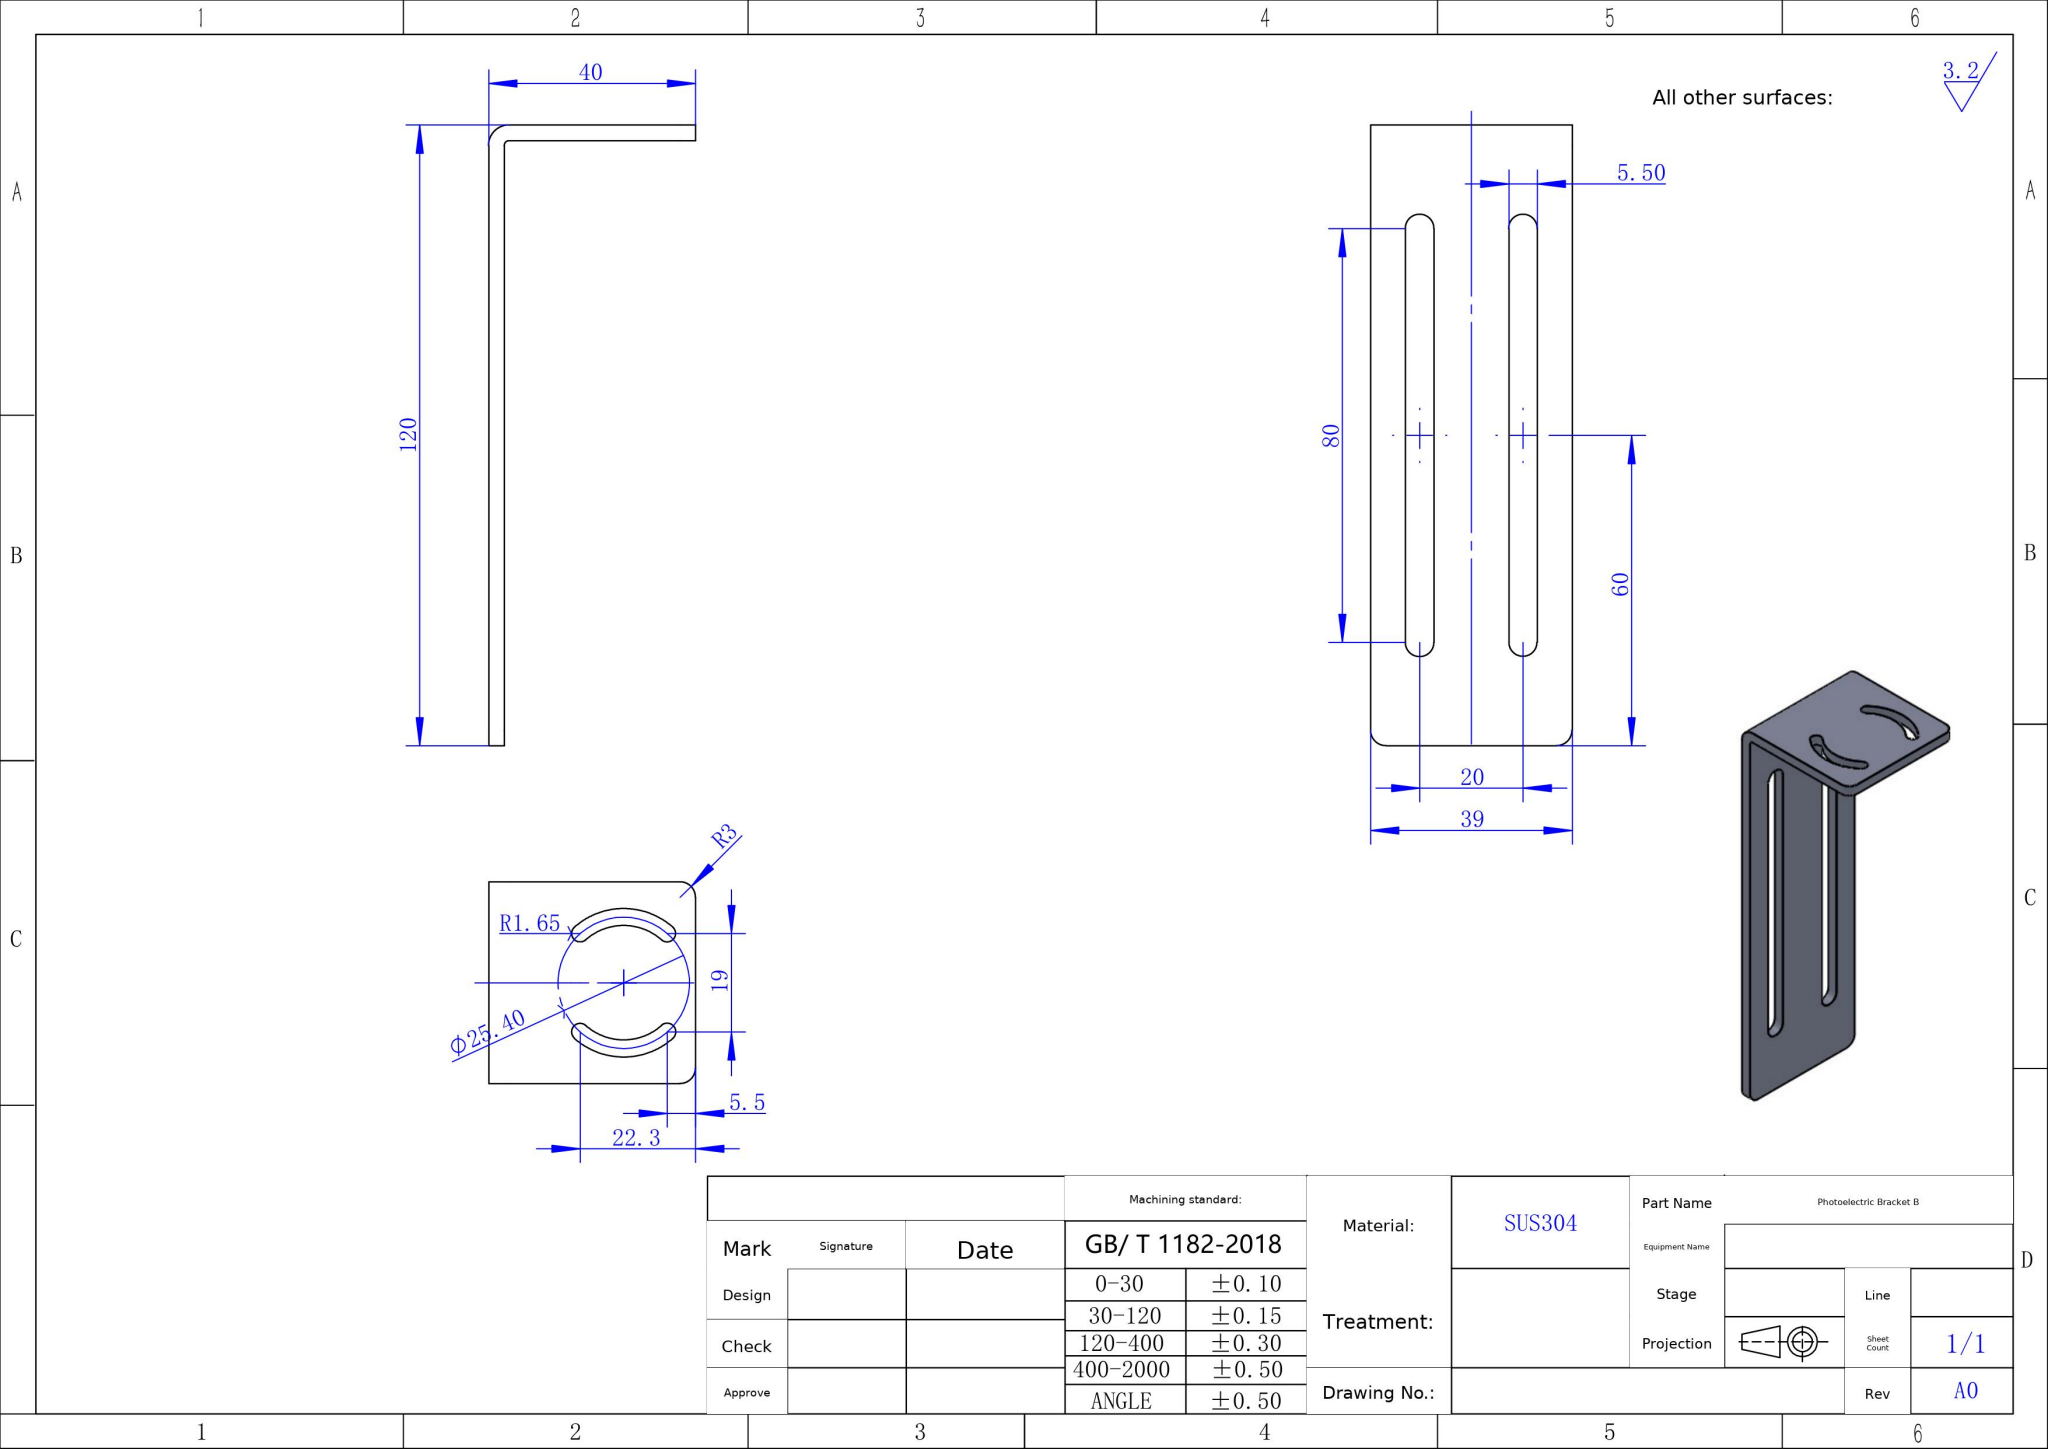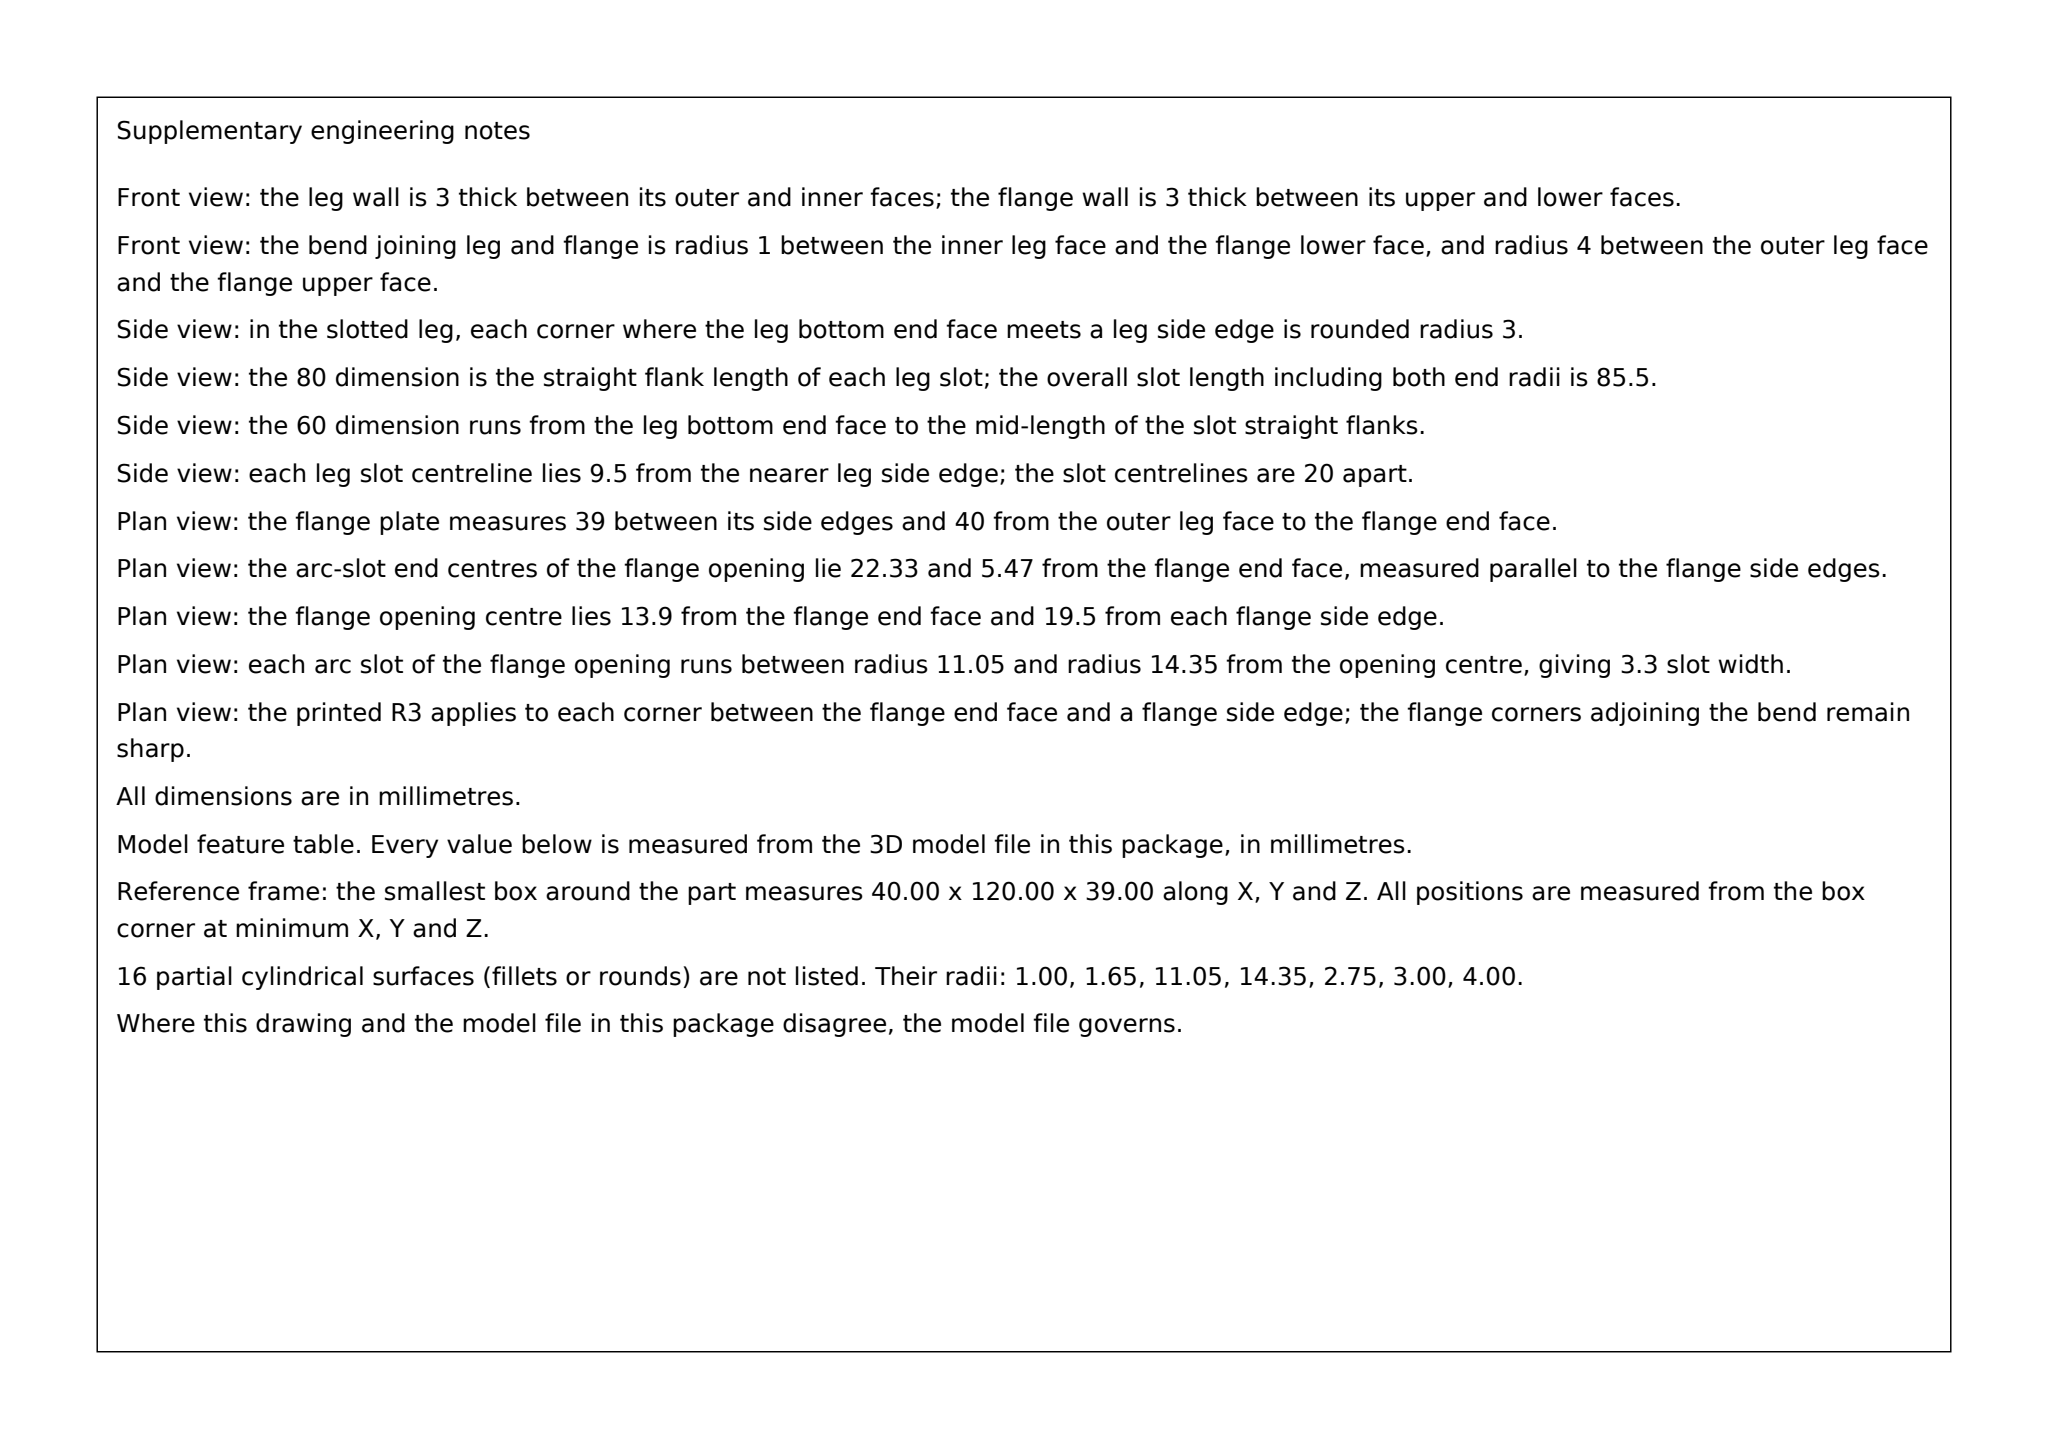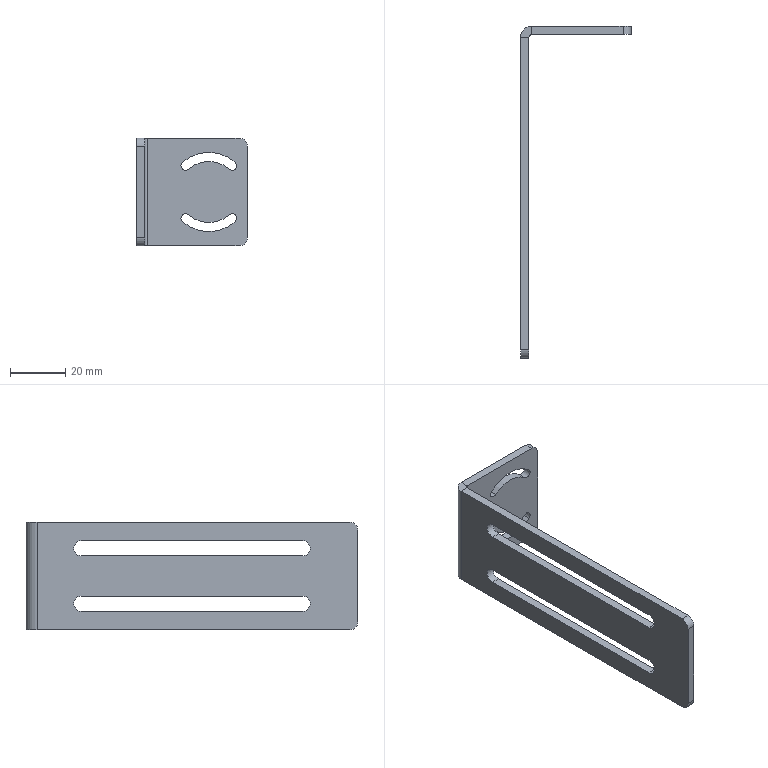Part | SolidWorks | mm | 1 solid | 36 faces | box 40 x 120 x 39 mm | volume 15021 mm3 | cylinder 20 | plane 16 | commonest cylinder face diameters 3.3 x6 6 x4 5.5 x4 28.7 x2 22.1 x2 8 x1 2 x1
Drawing notes:
SHEET MATL THK 3 TYP | from the solid: Planes x=0 & x=3 (vert leg), y=117 & y=120 (horiz plate): 3 mm wall
BEND AT L CORNER: INSIDE R1, OUTSIDE R4 | from the solid: Cylinders dia 2.0 and dia 8.0, axis z at (x=4.0, y=116.0), len 39
VERT LEG BOTTOM CORNERS R3 (2X) | from the solid: dia 6.0 cyl, axis x, at (y=3, z=3) and (y=3, z=36), len 3